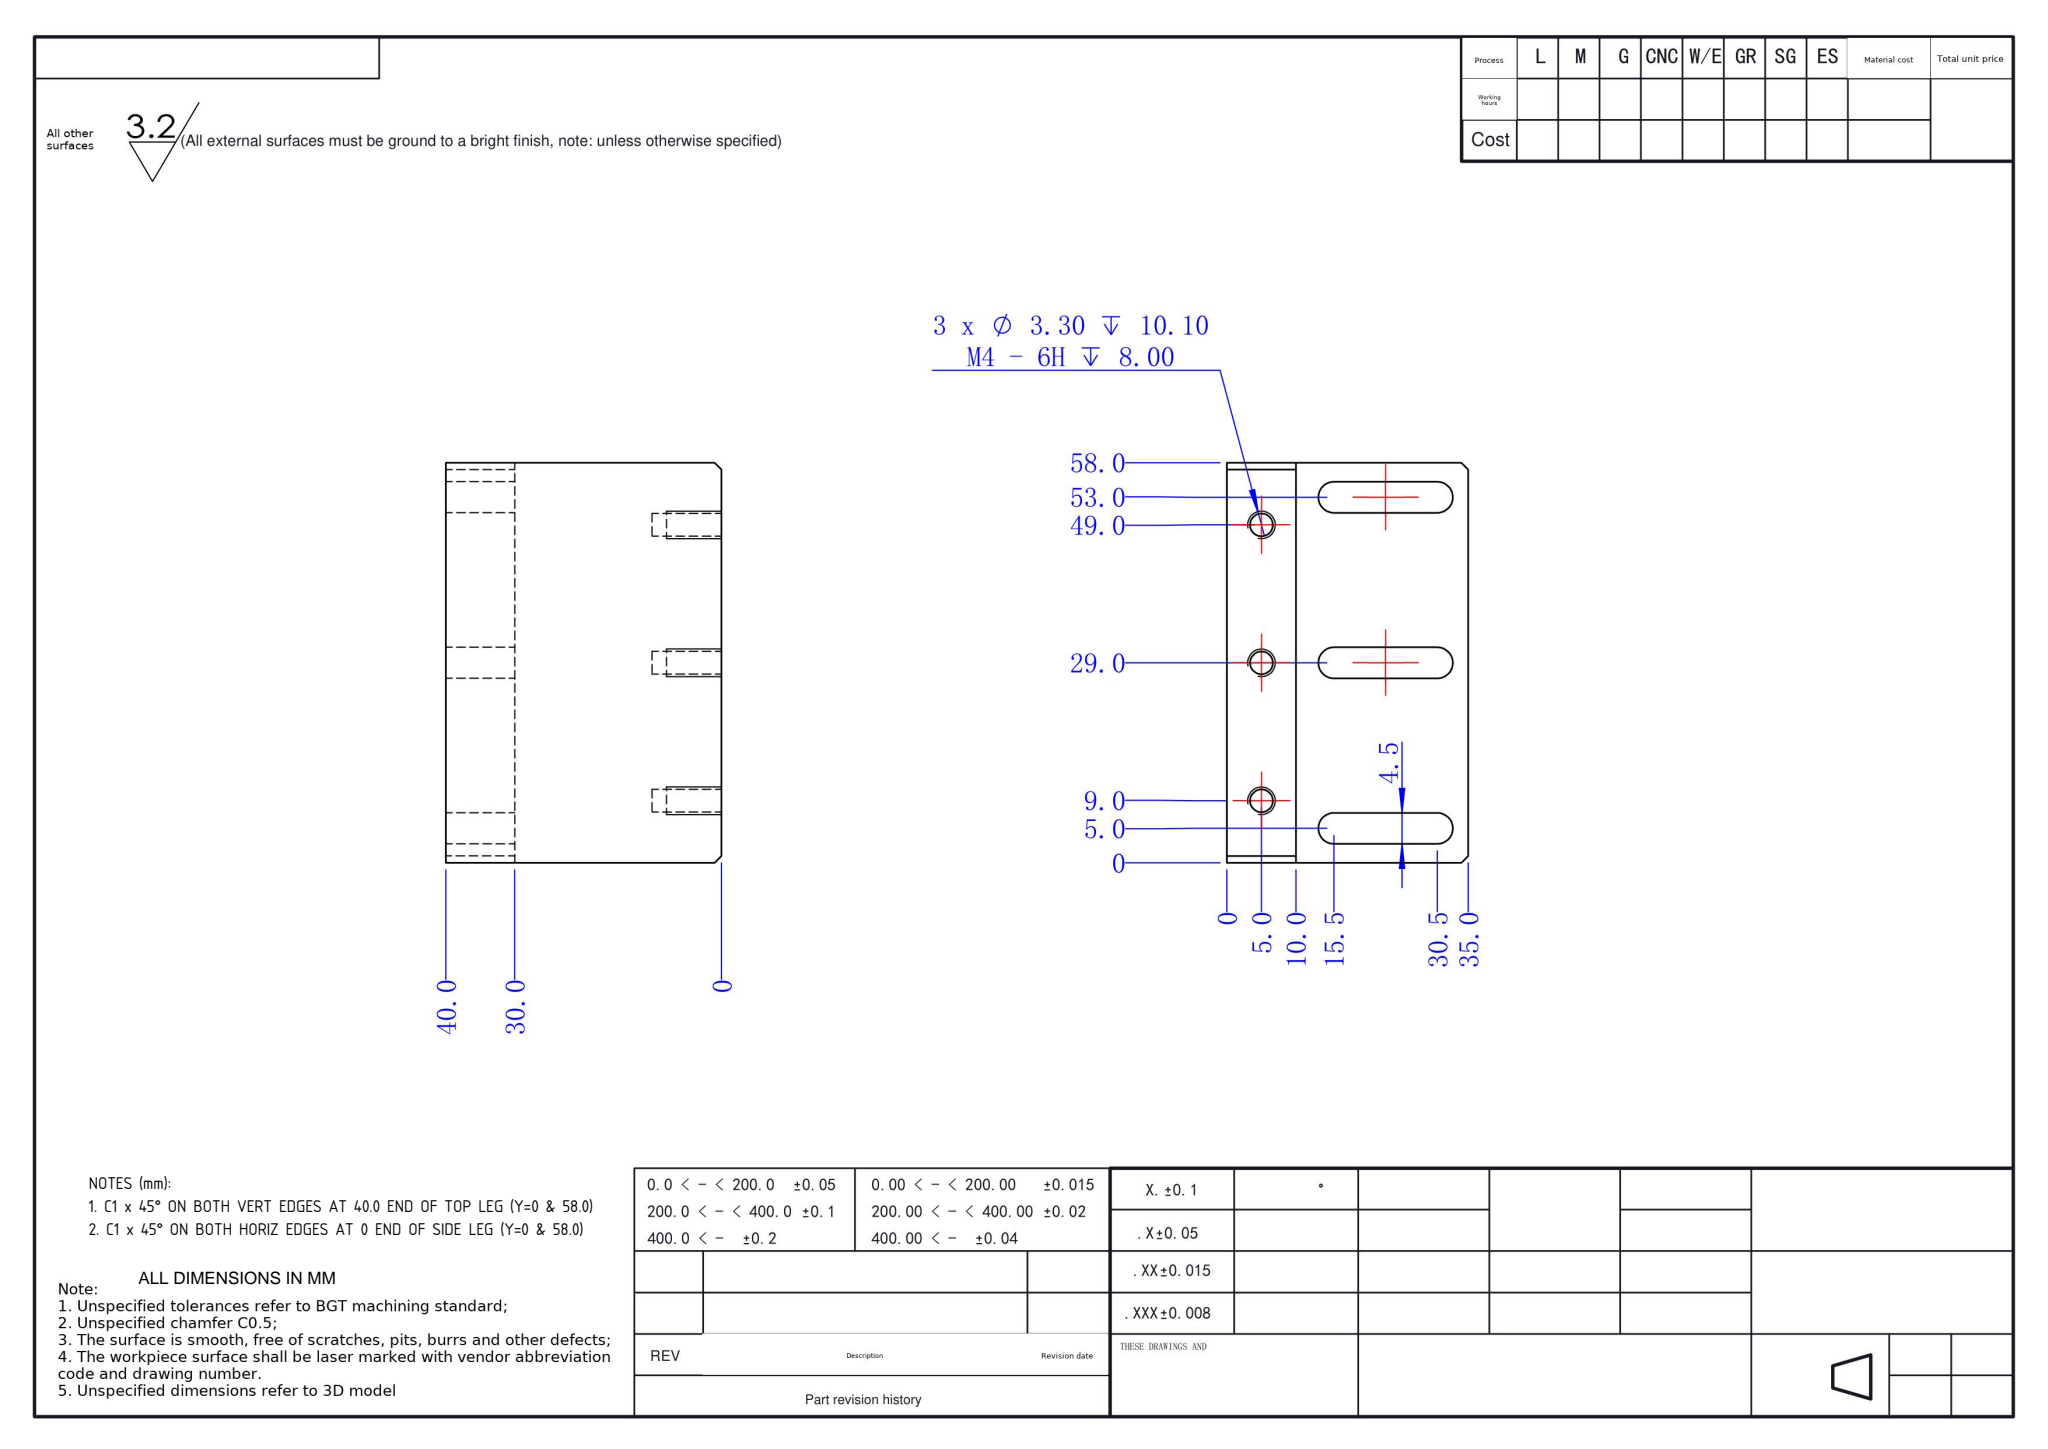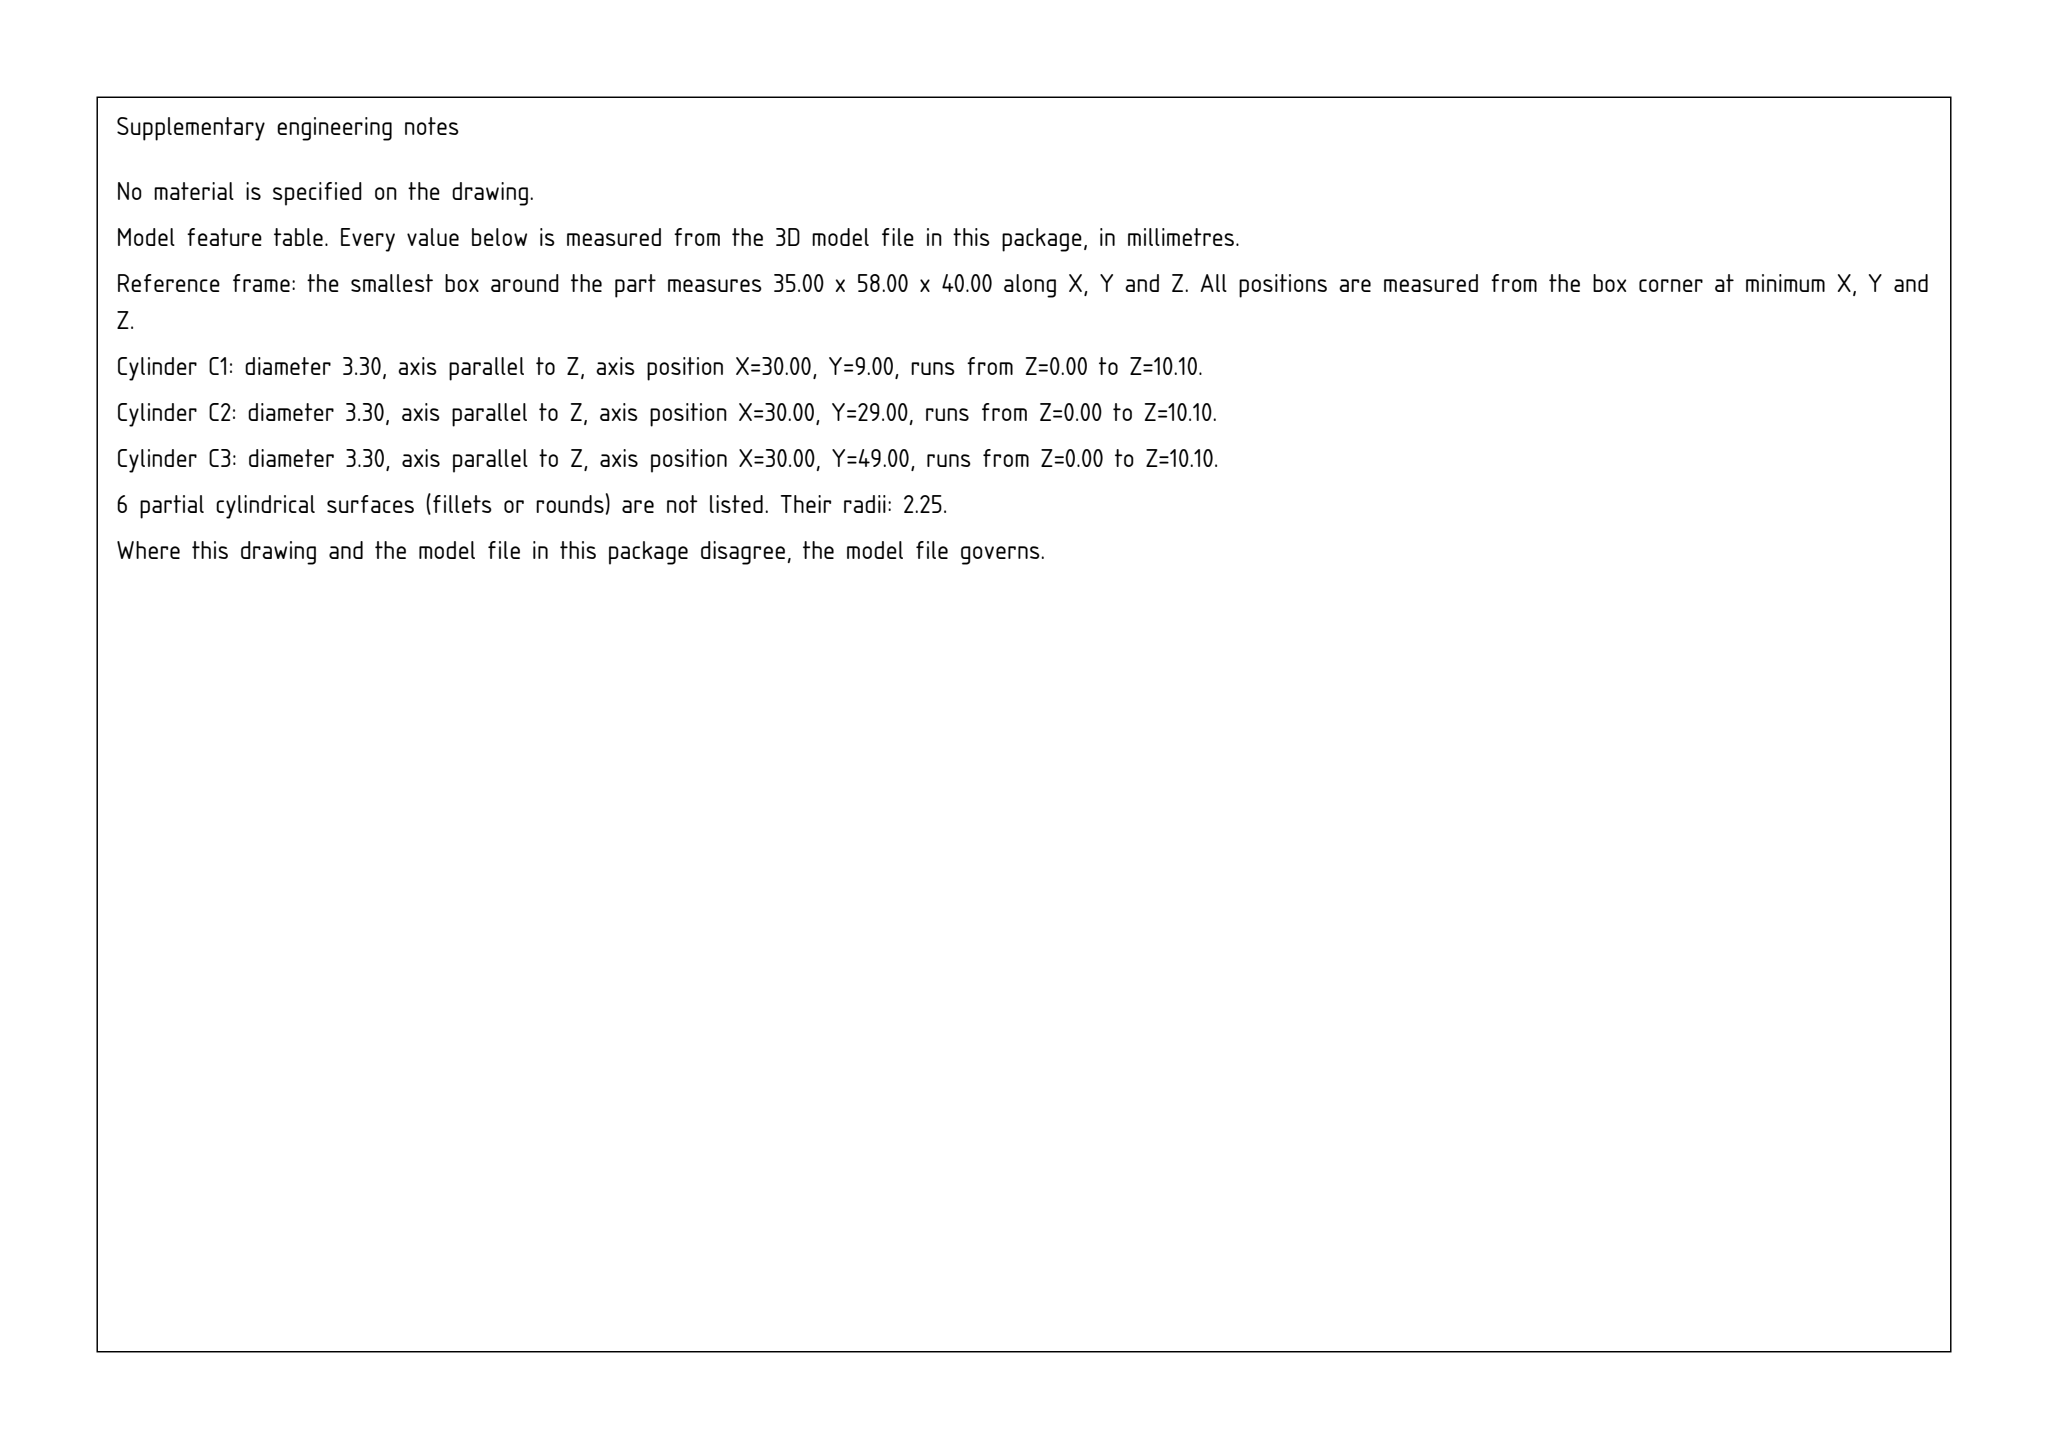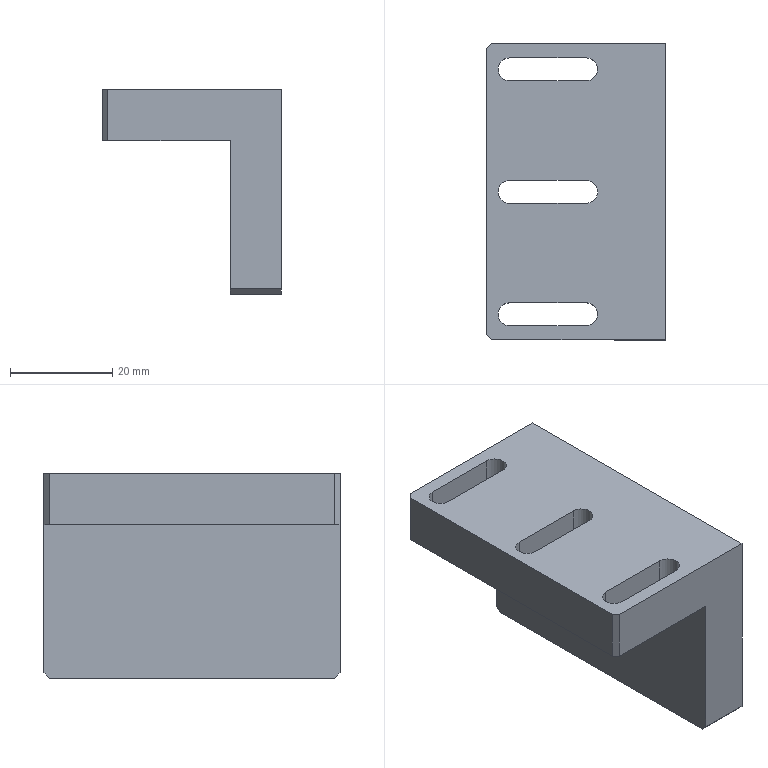Part | SolidWorks | mm | 1 solid | 36 faces | box 35 x 58 x 40 mm | volume 34919 mm3 | plane 21 | cylinder 15 | commonest cylinder face diameters 4.5 x9 3.3 x6
Drawing notes:
C1 x 45° ON BOTH VERT EDGES AT 40.0 END OF TOP LEG (Y=0 & 58.0) | from the solid: inclined_planes 45/45/90 at bbox_from [0,0,30] & [0,57,30], size 1x1x10
C1 x 45° ON BOTH HORIZ EDGES AT 0 END OF SIDE LEG (Y=0 & 58.0) | from the solid: inclined_planes 90/45/45 at bbox_from [25,0,0] & [25,57,0], size 10x1x1
build123d program:
from build123d import *

# Parameters (mm, degrees)
BOSS_EXTRUDE1_DEPTH   = 58
CUT_EXTRUDE1_DEPTH    = 75.088
CHAMFER1_SIZE         = 1
M4_TAPPED_HOLE1_D     = 3.3
M4_TAPPED_HOLE1_DEPTH = 10.1


with BuildPart() as part:
    # Sketch1 → Boss-Extrude1 (new body)
    with BuildSketch(Plane(origin=(0, 0, 0), x_dir=(1, 0, 0), z_dir=(0, 1, 0))):
        Polygon((0, 0), (0, 10), (25, 10), (25, 40), (35, 40), (35, 0), align=None)
    extrude(amount=BOSS_EXTRUDE1_DEPTH)

    # Sketch2 → Cut-Extrude1 (cut, through all)
    with BuildSketch(Plane(origin=(0, 0, -10), x_dir=(-1, 0, 0), z_dir=(0, 0, -1))):
        with BuildLine():
            Line((-4.5, 50.75), (-19.5, 50.75))
            ThreePointArc((-19.5, 50.75), (-21.75, 53), (-19.5, 55.25))
            Line((-19.5, 55.25), (-4.5, 55.25))
            ThreePointArc((-4.5, 55.25), (-2.25, 53), (-4.5, 50.75))
        make_face()
        with BuildLine():
            Line((-4.5, 26.75), (-19.5, 26.75))
            ThreePointArc((-19.5, 26.75), (-21.75, 29), (-19.5, 31.25))
            Line((-19.5, 31.25), (-4.5, 31.25))
            ThreePointArc((-4.5, 31.25), (-2.25, 29), (-4.5, 26.75))
        make_face()
        with BuildLine():
            Line((-19.5, 7.25), (-4.5, 7.25))
            ThreePointArc((-4.5, 7.25), (-2.25, 5), (-4.5, 2.75))
            Line((-4.5, 2.75), (-19.5, 2.75))
            ThreePointArc((-19.5, 2.75), (-21.75, 5), (-19.5, 7.25))
        make_face()
    extrude(amount=-CUT_EXTRUDE1_DEPTH, mode=Mode.SUBTRACT)

    # Chamfer1
    chamfer1_edges = [part.edges().sort_by_distance(p)[0] for p in [
        (30, 58, -40),
        (0, 58, -5),
        (0, 0, -5),
        (30, 0, -40),
    ]]
    chamfer(chamfer1_edges, length=CHAMFER1_SIZE)

    # M4 Tapped Hole1
    with Locations(Plane(origin=(0, 0, -40), x_dir=(-1, 0, 0), z_dir=(0, 0, -1))):
        with Locations((-30, 9), (-30, 29), (-30, 49)):
            Hole(M4_TAPPED_HOLE1_D / 2, depth=M4_TAPPED_HOLE1_DEPTH)


solid = part.part